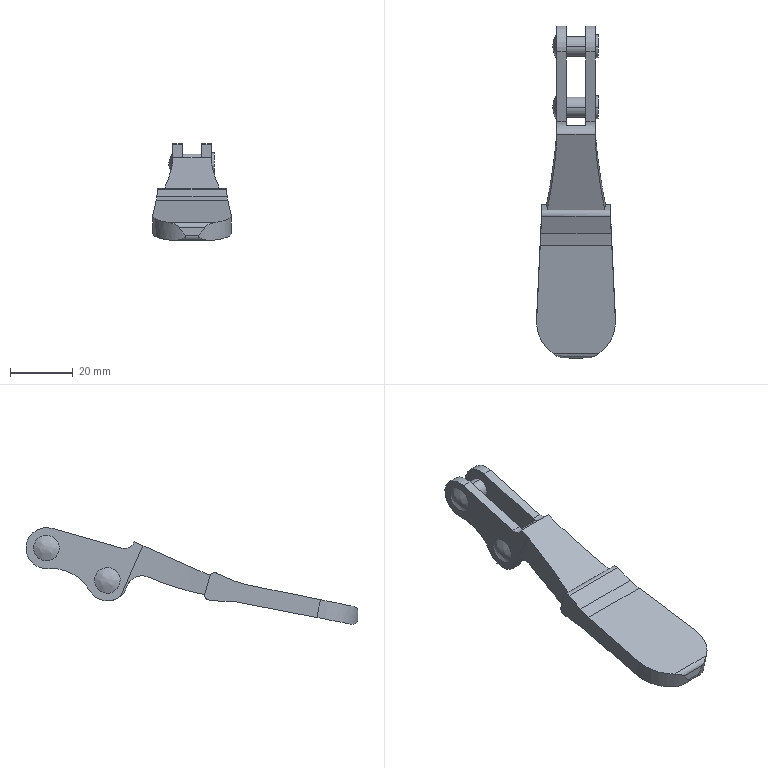Component | SolidWorks | AD12-MC01H-4_2_03.SDASM-1_AD12-_MC01H-4_h.sdprt-1 | 1 solid | 61 faces | volume 12016 mm3 | cylinder 34 | plane 25 | spline 2 | commonest cylinder face diameters 6.35 x4 7.35 x4 3.2 x4 383.016 x4 13 x4 25.026 x2 115.571 x2 9.979 x2